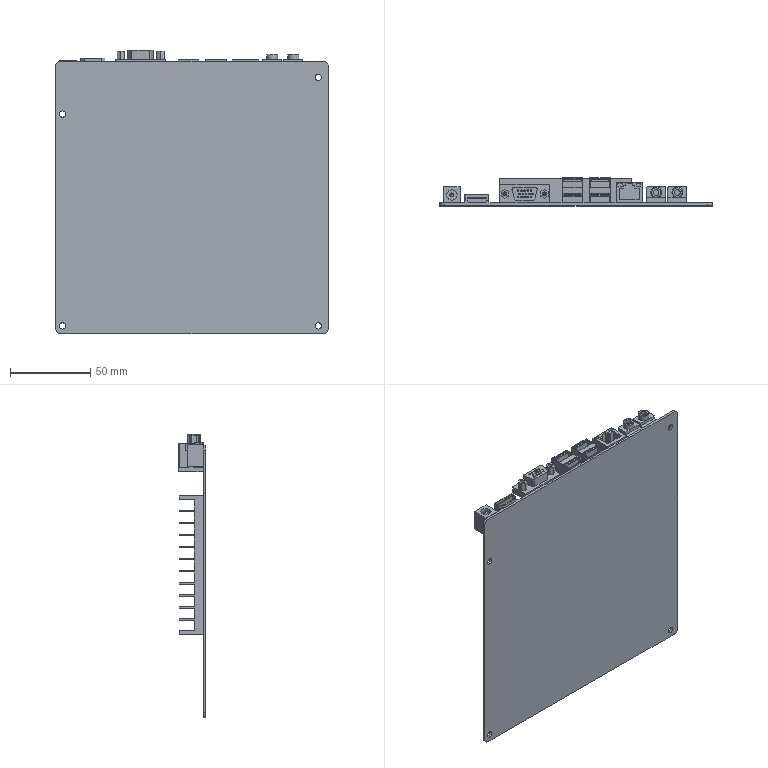Component | SolidWorks | 10.1InchMotherboard-1 | 1 solid | 326 faces | box 170 x 17.2 x 176.85 mm | volume 110739 mm3 | plane 241 | cylinder 71 | cone 8 | torus 4 | sphere 2 | commonest cylinder face diameters 1 x34 3.9 x8 2.5 x6 2 x5 3.5 x4 6.8 x4 1.5 x4 6 x4
build123d program:
from build123d import *

# Parameters (mm, degrees)
BOSS_EXTRUDE1_DEPTH   = 1.6
SKETCH2_R             = 1.95
CUT_EXTRUDE1_DEPTH    = 1.6
SKETCH3_W             = 82.4
SKETCH3_H             = 86.3
BOSS_EXTRUDE2_DEPTH   = 15.1
SKETCH4_W             = 82.4
SKETCH4_H             = 6.35
CUT_EXTRUDE2_DEPTH    = 9.6
SKETCH5_W             = 13
SKETCH5_H             = 17.5
BOSS_EXTRUDE3_DEPTH   = 15.6
SKETCH6_W             = 30.8
SKETCH6_H             = 4.5
BOSS_EXTRUDE4_DEPTH   = 11.3
BOSS_EXTRUDE5_DEPTH   = 5.85
BOSS_EXTRUDE6_DEPTH   = 5.4
SKETCH11_R            = 0.75
CUT_EXTRUDE3_DEPTH    = 5.4
M3_TAPPED_HOLE1_D     = 2.5
M3_TAPPED_HOLE1_DEPTH = 5
M3_TAPPED_HOLE1_TIP   = 0.7511
SKETCH14_R            = 0.5
CUT_EXTRUDE4_DEPTH    = 5.4
SKETCH15_W            = 12
SKETCH15_H            = 2.65
SKETCH15_W_2          = 11
SKETCH15_H_2          = 1.5
SKETCH15_H_3          = 3
CUT_EXTRUDE5_DEPTH    = 15
CHAMFER1_SIZE         = 0.3
SKETCH16_W            = 16.5
SKETCH16_H            = 16
BOSS_EXTRUDE7_DEPTH   = 13
CUT_EXTRUDE6_DEPTH    = 13
SKETCH18_W            = 3
SKETCH18_H            = 1.5
CUT_EXTRUDE7_DEPTH    = 1
SKETCH19_W            = 12
SKETCH19_H            = 11
BOSS_EXTRUDE8_DEPTH   = 10
FILLET1_R             = 0.5
SKETCH20_W            = 25.25
SKETCH20_H            = 3.2
CUT_EXTRUDE8_DEPTH    = 2
SKETCH21_R            = 3.4
BOSS_EXTRUDE9_DEPTH   = 3.5
SKETCH22_R            = 1.75
CUT_EXTRUDE9_DEPTH    = 10.5
FILLET2_R             = 0.5
SKETCH23_W            = 15
SKETCH23_H            = 12
BOSS_EXTRUDE10_DEPTH  = 5.6
CHAMFER2_SIZE         = 2
SKETCH24_W            = 12
SKETCH24_H            = 0.5
CUT_EXTRUDE10_DEPTH   = 10.6
SKETCH25_W            = 10.2
SKETCH25_H            = 13.25
BOSS_EXTRUDE11_DEPTH  = 10
SKETCH26_R            = 3.2
SKETCH26_R_2          = 1.25
CUT_EXTRUDE11_DEPTH   = 10
FILLET3_R             = 1.25


with BuildPart() as part:
    # Sketch1 → Boss-Extrude1 (new body)
    with BuildSketch(Plane(origin=(0, 0, 0), x_dir=(1, 0, 0), z_dir=(0, 1, 0))):
        with BuildLine():
            Line((-82, -85), (82, -85))
            ThreePointArc((82, -85), (84.121, -84.121), (85, -82))
            Line((85, -82), (85, 82))
            ThreePointArc((85, 82), (84.121, 84.121), (82, 85))
            Line((82, 85), (-82, 85))
            ThreePointArc((-82, 85), (-84.121, 84.121), (-85, 82))
            Line((-85, 82), (-85, -82))
            ThreePointArc((-85, -82), (-84.121, -84.121), (-82, -85))
        make_face()
    extrude(amount=BOSS_EXTRUDE1_DEPTH)

    # Sketch2 → Cut-Extrude1 (cut)
    with BuildSketch(Plane(origin=(0, 1.6, 0), x_dir=(1, 0, 0), z_dir=(0, 1, 0))):
        with Locations(Location((-80.8, 80.15, 0), (0, 0, 270))):
            Circle(SKETCH2_R)
        with Locations(Location((78.85, 80.15, 0), (0, 0, 270))):
            Circle(SKETCH2_R)
        with Locations(Location((78.85, -74.85, 0), (0, 0, 270))):
            Circle(SKETCH2_R)
        with Locations(Location((-80.8, -52.05, 0), (0, 0, 270))):
            Circle(SKETCH2_R)
    extrude(amount=-CUT_EXTRUDE1_DEPTH, mode=Mode.SUBTRACT)

    # Sketch3 → Boss-Extrude2 (add)
    with BuildSketch(Plane(origin=(0, 1.6, 0), x_dir=(1, 0, 0), z_dir=(0, 1, 0))):
        with Locations((-6.5, -10.25)):
            Rectangle(SKETCH3_W, SKETCH3_H)
    extrude(amount=BOSS_EXTRUDE2_DEPTH)

    # Sketch4 → Cut-Extrude2 (cut)
    with BuildSketch(Plane(origin=(0, 16.7, 0), x_dir=(1, 0, 0), z_dir=(0, 1, 0))):
        with Locations((-6.5, -2.75)):
            Rectangle(SKETCH4_W, SKETCH4_H)
        with Locations((-6.5, -10.25)):
            Rectangle(SKETCH4_W, SKETCH4_H)
        with Locations((-6.5, 4.75)):
            Rectangle(SKETCH4_W, SKETCH4_H)
        with Locations((-6.5, 12.25)):
            Rectangle(SKETCH4_W, SKETCH4_H)
        with Locations((-6.5, 19.75)):
            Rectangle(SKETCH4_W, SKETCH4_H)
        with Locations((-6.5, 27.25)):
            Rectangle(SKETCH4_W, SKETCH4_H)
        with Locations((-6.5, -17.75)):
            Rectangle(SKETCH4_W, SKETCH4_H)
        with Locations((-6.5, -25.25)):
            Rectangle(SKETCH4_W, SKETCH4_H)
        with Locations((-6.5, -32.75)):
            Rectangle(SKETCH4_W, SKETCH4_H)
        with Locations((-6.5, -40.25)):
            Rectangle(SKETCH4_W, SKETCH4_H)
        with Locations((-6.5, -47.75)):
            Rectangle(SKETCH4_W, SKETCH4_H)
    extrude(amount=-CUT_EXTRUDE2_DEPTH, mode=Mode.SUBTRACT)

    # Sketch5 → Boss-Extrude3 (add)
    with BuildSketch(Plane(origin=(0, 1.6, 0), x_dir=(1, 0, 0), z_dir=(0, 1, 0))):
        with Locations((-2.2, -77.25)):
            Rectangle(SKETCH5_W, SKETCH5_H)
        with Locations((15, -77.25)):
            Rectangle(SKETCH5_W, SKETCH5_H)
    extrude(amount=BOSS_EXTRUDE3_DEPTH)

    # Sketch6 → Boss-Extrude4 (add)
    with BuildSketch(Plane(origin=(0, 1.6, 0), x_dir=(1, 0, 0), z_dir=(0, 1, 0))):
        with Locations((-32.1, -83.75)):
            Rectangle(SKETCH6_W, SKETCH6_H)
    extrude(amount=BOSS_EXTRUDE4_DEPTH)

    # Sketch7 → Boss-Extrude5 (add)
    with BuildSketch(Plane.XY.offset(86)):
        with BuildLine():
            Line((-39.912, 9.972), (-38.531, 4.072))
            ThreePointArc((-38.531, 4.072), (-38.178, 3.516), (-37.557, 3.3))
            Line((-37.557, 3.3), (-26.643, 3.3))
            ThreePointArc((-26.643, 3.3), (-26.022, 3.516), (-25.669, 4.072))
            Line((-25.669, 4.072), (-24.288, 9.972))
            ThreePointArc((-24.288, 9.972), (-24.478, 10.821), (-25.261, 11.2))
            Line((-25.261, 11.2), (-38.939, 11.2))
            ThreePointArc((-38.939, 11.2), (-39.722, 10.821), (-39.912, 9.972))
        make_face()
    extrude(amount=BOSS_EXTRUDE5_DEPTH)

    # Sketch8 → Boss-Extrude6 (add)
    with BuildSketch(Plane.XY.offset(86)):
        Polygon((-44.425, 9.992), (-46.8, 8.621), (-46.8, 5.879), (-44.425, 4.508), (-42.05, 5.879), (-42.05, 8.621), align=None)
        Polygon((-19.775, 9.992), (-22.15, 8.621), (-22.15, 5.879), (-19.775, 4.508), (-17.4, 5.879), (-17.4, 8.621), align=None)
    extrude(amount=BOSS_EXTRUDE6_DEPTH)

    # Sketch11 → Cut-Extrude3 (cut)
    with BuildSketch(Plane.XY.offset(91.4)):
        with Locations((-44.425, 7.25)):
            Circle(SKETCH11_R)
        with Locations((-19.775, 7.25)):
            Circle(SKETCH11_R)
    extrude(amount=-CUT_EXTRUDE3_DEPTH, mode=Mode.SUBTRACT)

    # M3 Tapped Hole1
    with Locations(Plane.XY.offset(91.4)):
        with Locations((-44.425, 7.25), (-19.775, 7.25)):
            Hole(M3_TAPPED_HOLE1_D / 2, depth=M3_TAPPED_HOLE1_DEPTH)
            with Locations((0, 0, -(M3_TAPPED_HOLE1_DEPTH + M3_TAPPED_HOLE1_TIP / 2))):  # 118° drill point
                Cone(0, M3_TAPPED_HOLE1_D / 2, M3_TAPPED_HOLE1_TIP, mode=Mode.SUBTRACT)

    # Sketch14 → Cut-Extrude4 (cut)
    with BuildSketch(Plane.XY.offset(91.85)):
        with Locations((-32.1, 5.25)):
            Circle(SKETCH14_R)
        with Locations((-30.1, 5.25)):
            Circle(SKETCH14_R)
        with Locations((-28.1, 5.25)):
            Circle(SKETCH14_R)
        with Locations((-34.1, 5.25)):
            Circle(SKETCH14_R)
        with Locations((-36.1, 5.25)):
            Circle(SKETCH14_R)
        with Locations((-28.1, 9.25)):
            Circle(SKETCH14_R)
        with Locations((-30.1, 9.25)):
            Circle(SKETCH14_R)
        with Locations((-34.1, 9.25)):
            Circle(SKETCH14_R)
        with Locations((-32.1, 9.25)):
            Circle(SKETCH14_R)
        with Locations((-36.1, 9.25)):
            Circle(SKETCH14_R)
        with Locations((-31.1, 7.25)):
            Circle(SKETCH14_R)
        with Locations((-29.1, 7.25)):
            Circle(SKETCH14_R)
        with Locations((-27.1, 7.25)):
            Circle(SKETCH14_R)
        with Locations((-33.1, 7.25)):
            Circle(SKETCH14_R)
        with Locations((-35.1, 7.25)):
            Circle(SKETCH14_R)
    extrude(amount=-CUT_EXTRUDE4_DEPTH, mode=Mode.SUBTRACT)

    # Sketch15 → Cut-Extrude5 (cut)
    # profile 1 of 8: a face of its own
    with BuildSketch(Plane.XY.offset(86)):
        with Locations((-2.2, 15.375)):
            Rectangle(SKETCH15_W, SKETCH15_H)
        with Locations((-2.2, 15.55)):
            Rectangle(SKETCH15_W_2, SKETCH15_H_2, mode=Mode.SUBTRACT)
    # profile 2 of 8: a face of its own
    with BuildSketch(Plane.XY.offset(86)):
        with Locations((-2.2, 12.55)):
            Rectangle(SKETCH15_W, SKETCH15_H_3)
    # profile 3 of 8: a face of its own
    with BuildSketch(Plane.XY.offset(86)):
        with Locations((-2.2, 6.425)):
            Rectangle(SKETCH15_W, SKETCH15_H)
        with Locations((-2.2, 6.5)):
            Rectangle(SKETCH15_W_2, SKETCH15_H_2, mode=Mode.SUBTRACT)
    # profile 4 of 8: a face of its own
    with BuildSketch(Plane.XY.offset(86)):
        with Locations((-2.2, 3.6)):
            Rectangle(SKETCH15_W, SKETCH15_H_3)
    # profile 5 of 8: a face of its own
    with BuildSketch(Plane.XY.offset(86)):
        with Locations((15, 15.375)):
            Rectangle(SKETCH15_W, SKETCH15_H)
        with Locations((15, 15.55)):
            Rectangle(SKETCH15_W_2, SKETCH15_H_2, mode=Mode.SUBTRACT)
    # profile 6 of 8: a face of its own
    with BuildSketch(Plane.XY.offset(86)):
        with Locations((15, 12.55)):
            Rectangle(SKETCH15_W, SKETCH15_H_3)
    # profile 7 of 8: a face of its own
    with BuildSketch(Plane.XY.offset(86)):
        with Locations((15, 6.425)):
            Rectangle(SKETCH15_W, SKETCH15_H)
        with Locations((15, 6.5)):
            Rectangle(SKETCH15_W_2, SKETCH15_H_2, mode=Mode.SUBTRACT)
    # profile 8 of 8: a face of its own
    with BuildSketch(Plane.XY.offset(86)):
        with Locations((15, 3.6)):
            Rectangle(SKETCH15_W, SKETCH15_H_3)
    extrude(amount=-CUT_EXTRUDE5_DEPTH, mode=Mode.SUBTRACT)

    # Chamfer1
    chamfer1_edges = [part.edges().sort_by_distance(p)[0] for p in [
        (-7.7, 15.55, 86),
        (-2.2, 14.8, 86),
        (-2.2, 16.3, 86),
        (3.3, 15.55, 86),
        (-7.7, 6.5, 86),
        (-2.2, 5.75, 86),
        (-2.2, 7.25, 86),
        (3.3, 6.5, 86),
        (9.5, 15.55, 86),
        (15, 14.8, 86),
        (15, 16.3, 86),
        (20.5, 15.55, 86),
        (9.5, 6.5, 86),
        (15, 5.75, 86),
        (15, 7.25, 86),
        (20.5, 6.5, 86),
    ]]
    chamfer(chamfer1_edges, length=CHAMFER1_SIZE)

    # Sketch16 → Boss-Extrude7 (add)
    with BuildSketch(Plane(origin=(0, 1.6, 0), x_dir=(1, 0, 0), z_dir=(0, 1, 0))):
        with Locations((33.25, -78)):
            Rectangle(SKETCH16_W, SKETCH16_H)
    extrude(amount=BOSS_EXTRUDE7_DEPTH)

    # Sketch17 → Cut-Extrude6 (cut)
    with BuildSketch(Plane.XY.offset(86)):
        Polygon((27.1, 3.9), (39.4, 3.9), (39.4, 10.8), (36.58, 10.8), (36.58, 12.4), (35.3, 12.4), (35.3, 13.8), (31.2, 13.8), (31.2, 12.4), (29.92, 12.4), (29.92, 10.8), (27.1, 10.8), align=None)
    extrude(amount=-CUT_EXTRUDE6_DEPTH, mode=Mode.SUBTRACT)

    # Sketch18 → Cut-Extrude7 (cut)
    with BuildSketch(Plane.XY.offset(86)):
        with Locations((27.5, 12.85)):
            Rectangle(SKETCH18_W, SKETCH18_H)
        with Locations((39, 12.85)):
            Rectangle(SKETCH18_W, SKETCH18_H)
    extrude(amount=-CUT_EXTRUDE7_DEPTH, mode=Mode.SUBTRACT)

    # Sketch19 → Boss-Extrude8 (add)
    with BuildSketch(Plane(origin=(0, 1.6, 0), x_dir=(1, 0, 0), z_dir=(0, 1, 0))):
        with Locations((50, -80.5)):
            Rectangle(SKETCH19_W, SKETCH19_H)
        with Locations((63.25, -80.5)):
            Rectangle(SKETCH19_W, SKETCH19_H)
    extrude(amount=BOSS_EXTRUDE8_DEPTH)

    # Fillet1
    fillet1_edges = [part.edges().sort_by_distance(p)[0] for p in [
        (56, 11.6, 80.5),
        (44, 11.6, 80.5),
        (69.25, 11.6, 80.5),
        (57.25, 11.6, 80.5),
    ]]
    fillet(fillet1_edges, radius=FILLET1_R)

    # Sketch20 → Cut-Extrude8 (cut)
    with BuildSketch(Plane.XY.offset(86)):
        with Locations((56.625, 3.2)):
            Rectangle(SKETCH20_W, SKETCH20_H)
    extrude(amount=-CUT_EXTRUDE8_DEPTH, mode=Mode.SUBTRACT)

    # Sketch21 → Boss-Extrude9 (add)
    with BuildSketch(Plane.XY.offset(86)):
        with Locations(Location((50, 8.2, 0), (0, 0, 270))):
            Circle(SKETCH21_R)
        with Locations(Location((63.25, 8.2, 0), (0, 0, 270))):
            Circle(SKETCH21_R)
    extrude(amount=BOSS_EXTRUDE9_DEPTH)

    # Sketch22 → Cut-Extrude9 (cut)
    with BuildSketch(Plane.XY.offset(89.5)):
        with Locations((50, 8.2)):
            Circle(SKETCH22_R)
        with Locations((63.25, 8.2)):
            Circle(SKETCH22_R)
    extrude(amount=-CUT_EXTRUDE9_DEPTH, mode=Mode.SUBTRACT)

    # Fillet2
    fillet2_edges = [part.edges().sort_by_distance(p)[0] for p in [
        (50, 11.6, 89.5),
        (63.25, 11.6, 89.5),
    ]]
    fillet(fillet2_edges, radius=FILLET2_R)

    # Sketch23 → Boss-Extrude10 (add)
    with BuildSketch(Plane(origin=(0, 1.6, 0), x_dir=(1, 0, 0), z_dir=(0, 1, 0))):
        with Locations((-61.85, -81)):
            Rectangle(SKETCH23_W, SKETCH23_H)
    extrude(amount=BOSS_EXTRUDE10_DEPTH)

    # Chamfer2
    chamfer2_edges = [part.edges().sort_by_distance(p)[0] for p in [
        (-54.35, 1.6, 86),
        (-69.35, 1.6, 86),
    ]]
    chamfer(chamfer2_edges, length=CHAMFER2_SIZE)

    # Sketch24 → Cut-Extrude10 (cut)
    with BuildSketch(Plane.XY.offset(87)):
        Polygon((-68.85, 6.7), (-68.85, 3.807), (-67.143, 2.1), (-56.557, 2.1), (-54.85, 3.807), (-54.85, 6.7), align=None)
        with Locations((-61.85, 4.95)):
            Rectangle(SKETCH24_W, SKETCH24_H, mode=Mode.SUBTRACT)
    extrude(amount=-CUT_EXTRUDE10_DEPTH, mode=Mode.SUBTRACT)

    # Sketch25 → Boss-Extrude11 (add)
    with BuildSketch(Plane(origin=(0, 1.6, 0), x_dir=(1, 0, 0), z_dir=(0, 1, 0))):
        with Locations((-77.45, -78.575)):
            Rectangle(SKETCH25_W, SKETCH25_H)
    extrude(amount=BOSS_EXTRUDE11_DEPTH)

    # Sketch26 → Cut-Extrude11 (cut)
    with BuildSketch(Plane.XY.offset(85.2)):
        with Locations((-77.45, 6.6)):
            Circle(SKETCH26_R)
        with Locations((-77.45, 6.6)):
            Circle(SKETCH26_R_2, mode=Mode.SUBTRACT)
    extrude(amount=-CUT_EXTRUDE11_DEPTH, mode=Mode.SUBTRACT)

    # Fillet3
    fillet3_edges = [part.edges().sort_by_distance(p)[0] for p in [
        (-78.7, 6.6, 85.2),
    ]]
    fillet(fillet3_edges, radius=FILLET3_R)


solid = part.part

# Placed as in the assembly
solid = solid.moved(Location((1138.486, 1497.312, 1981.133), (0, 0, 0)))